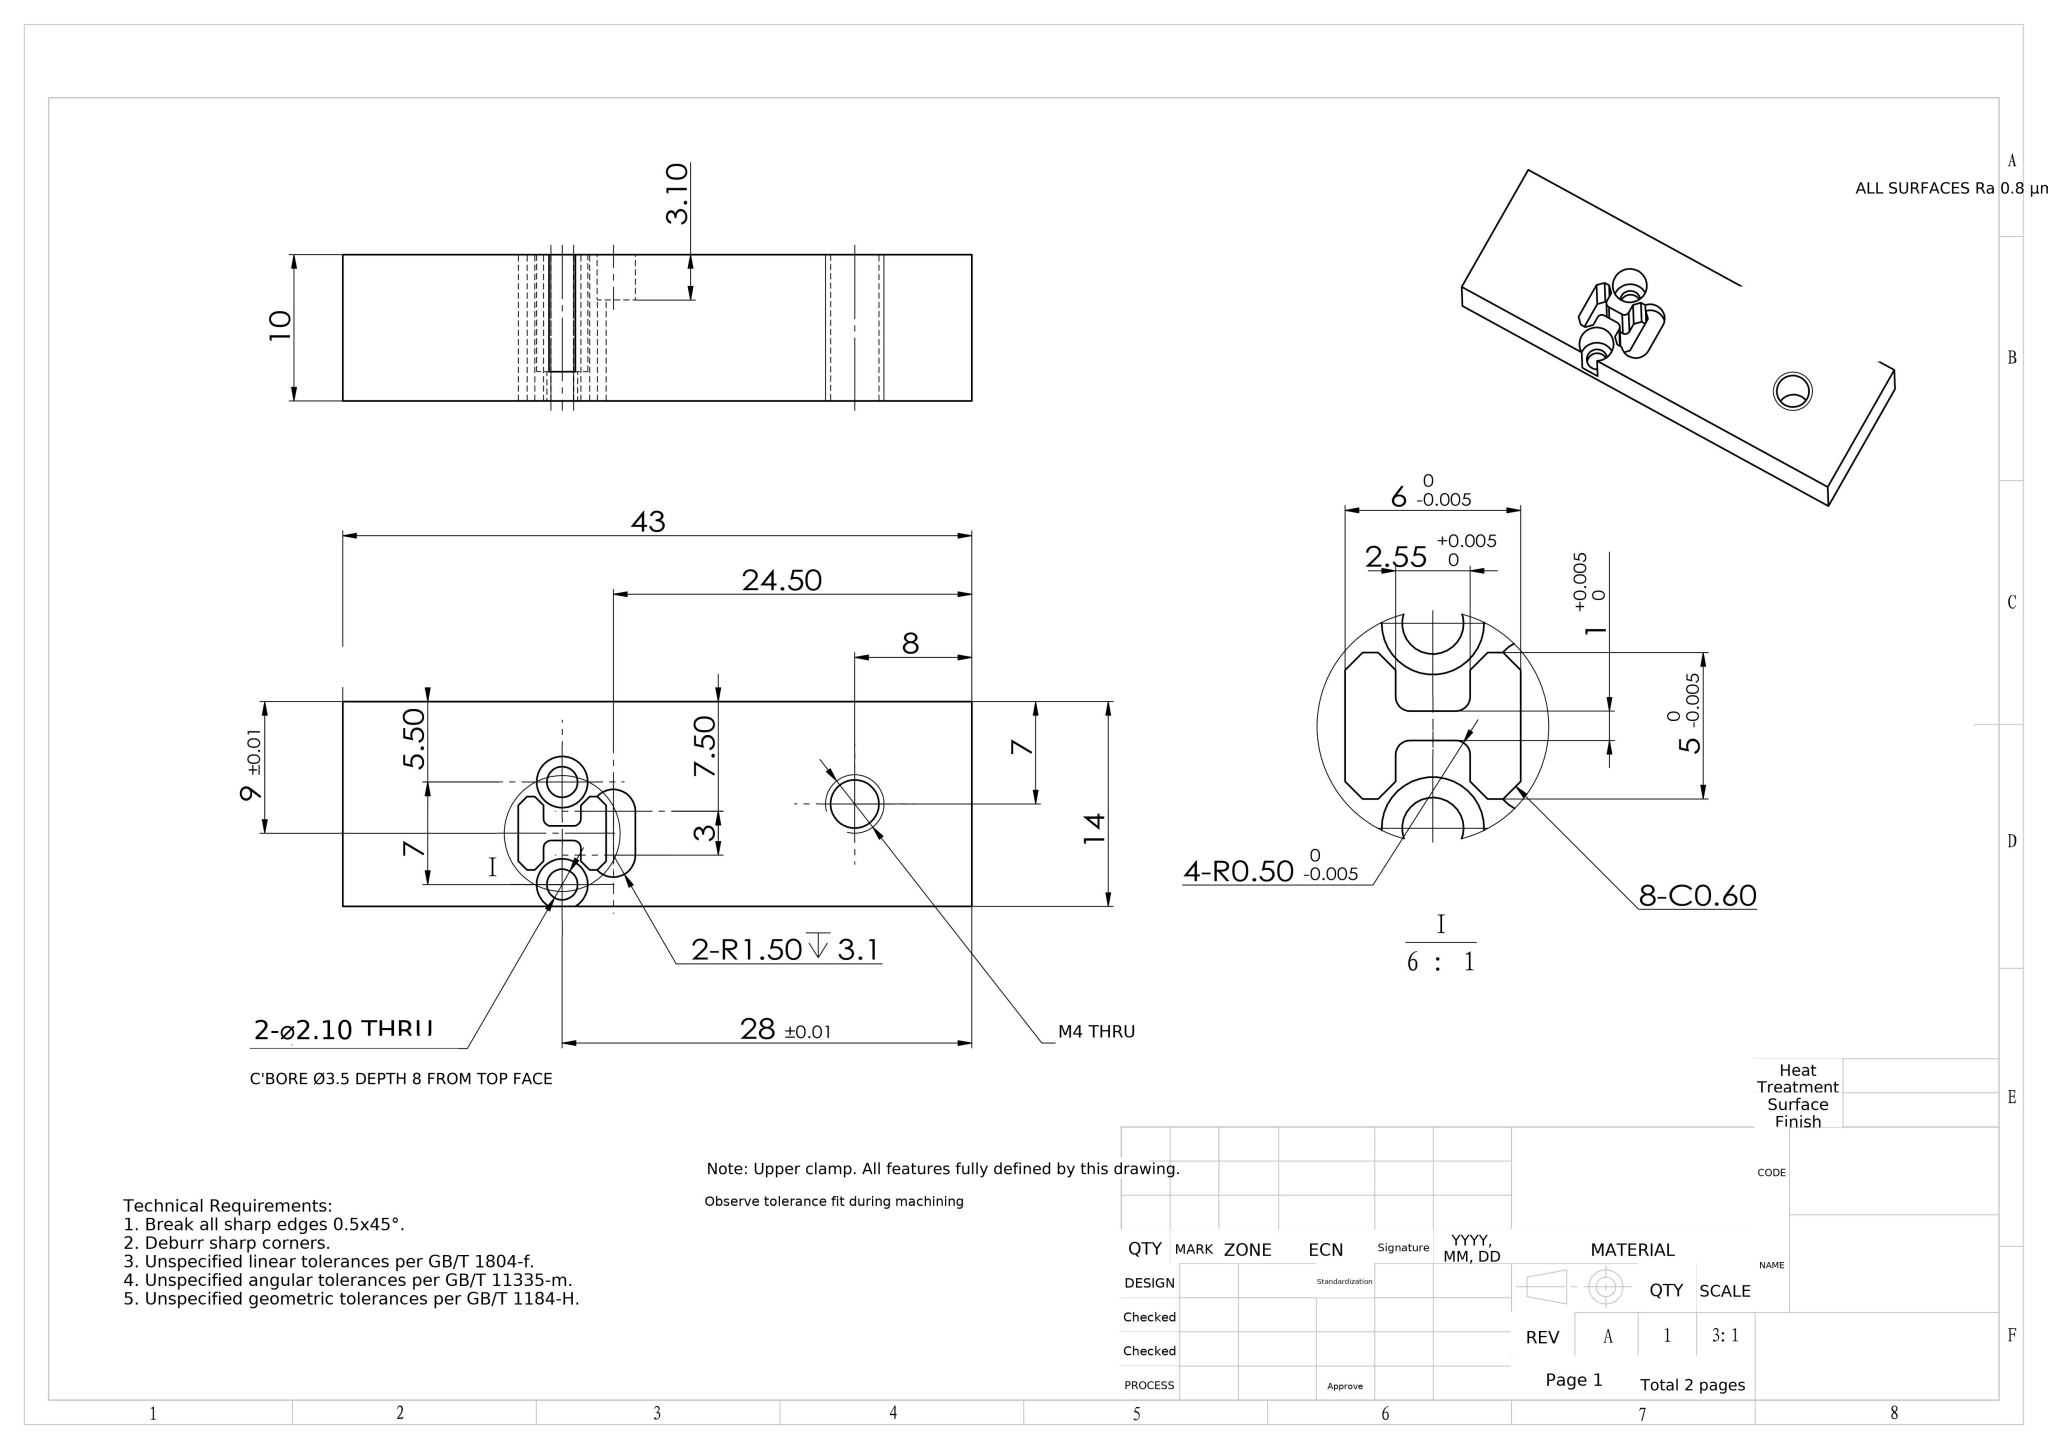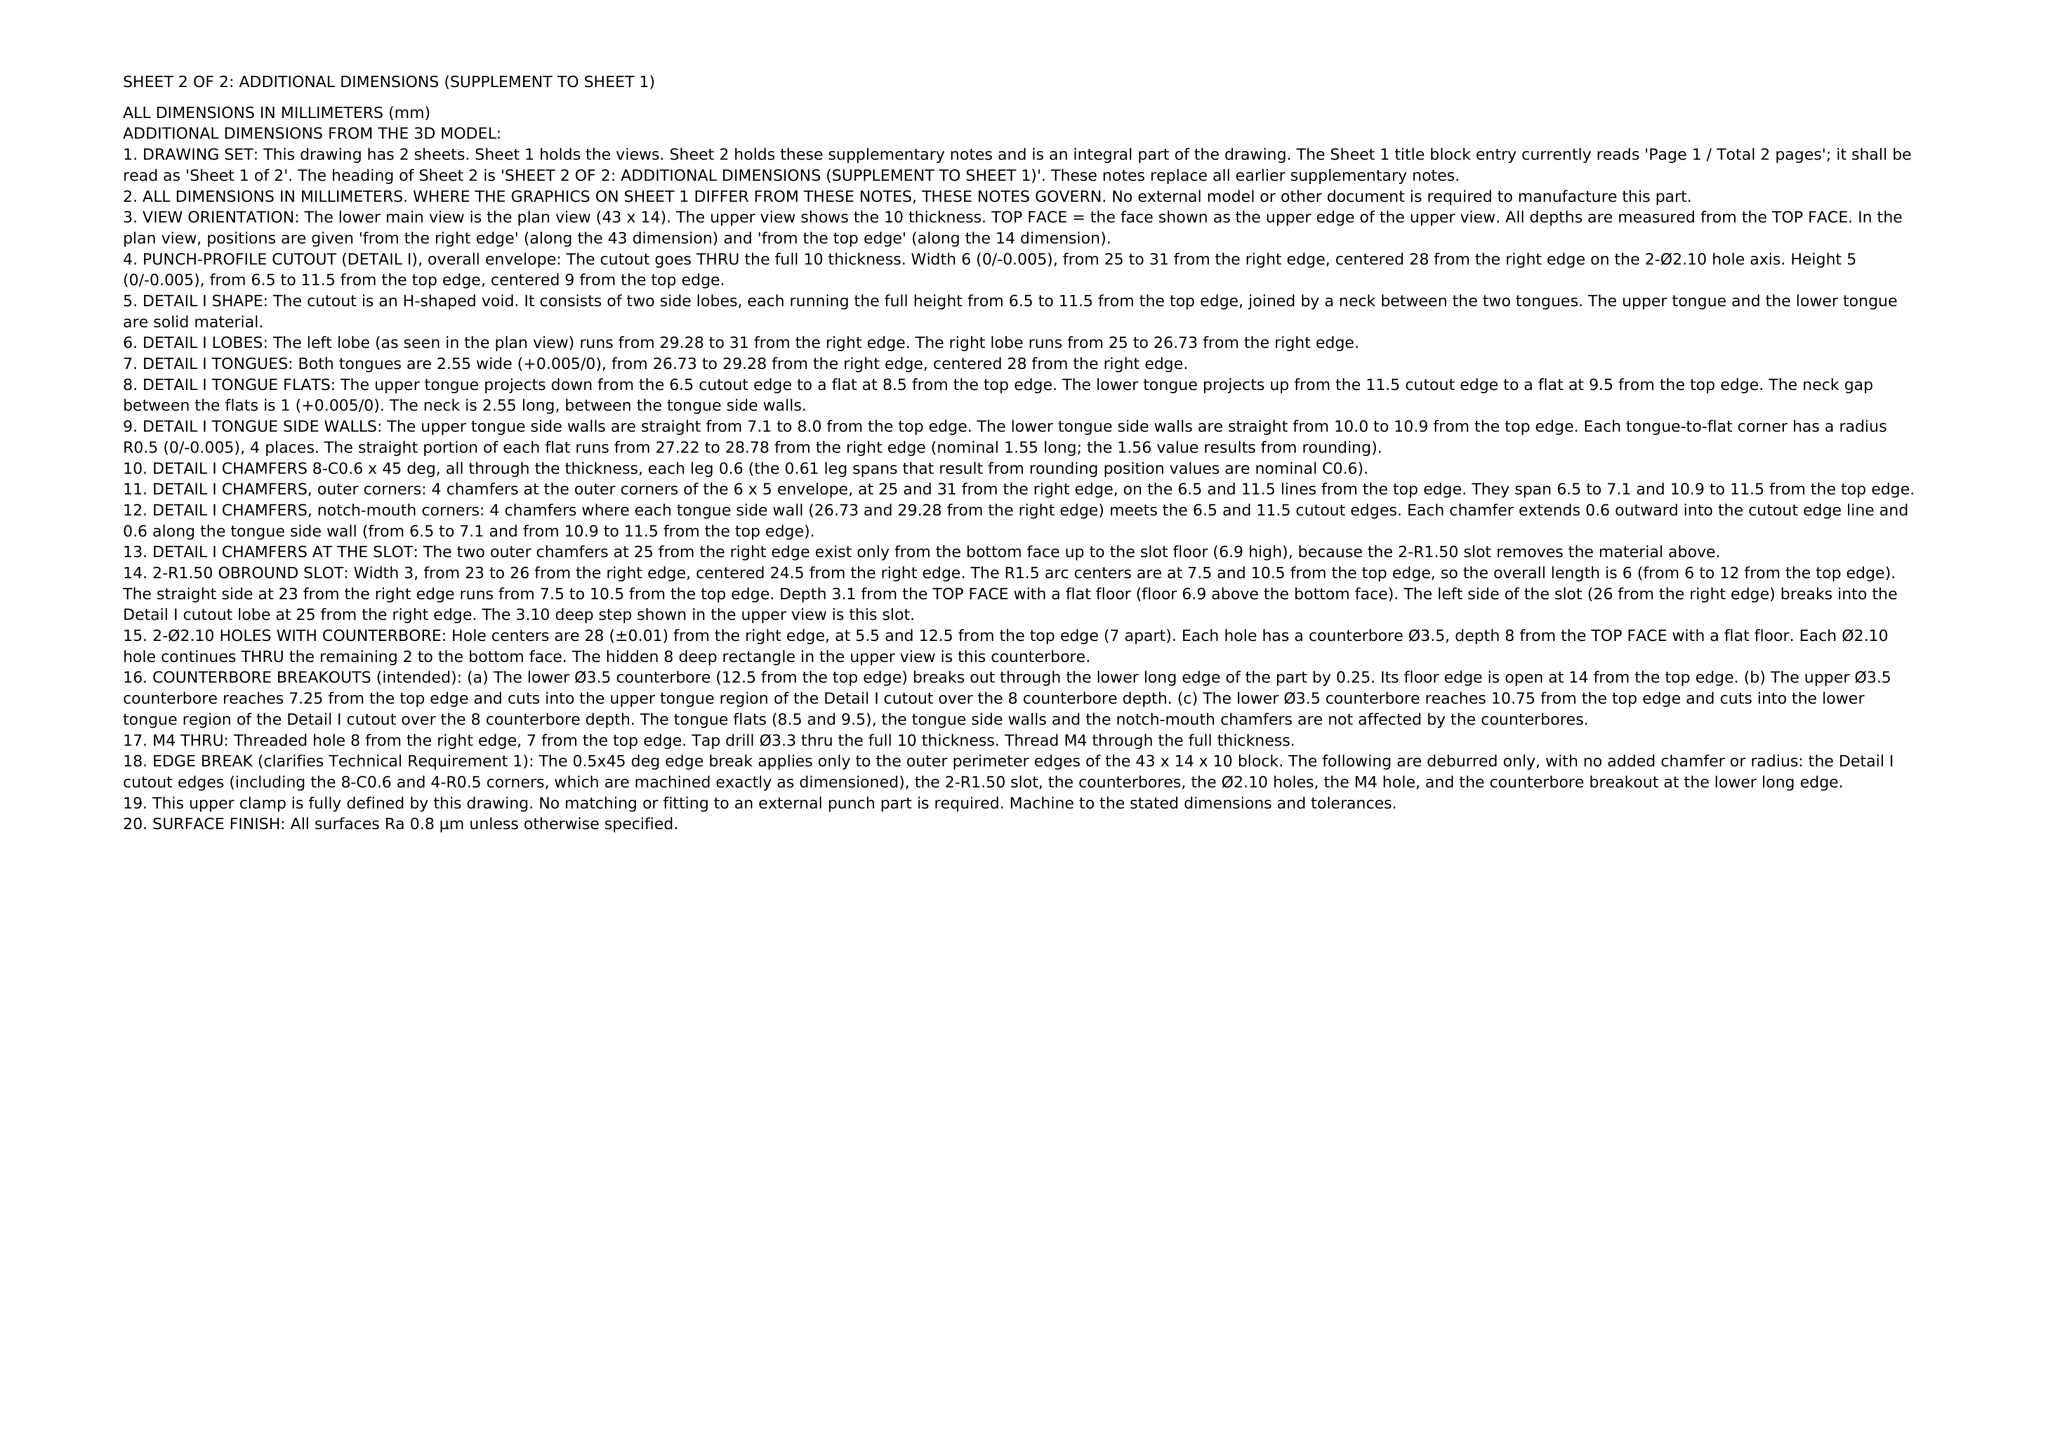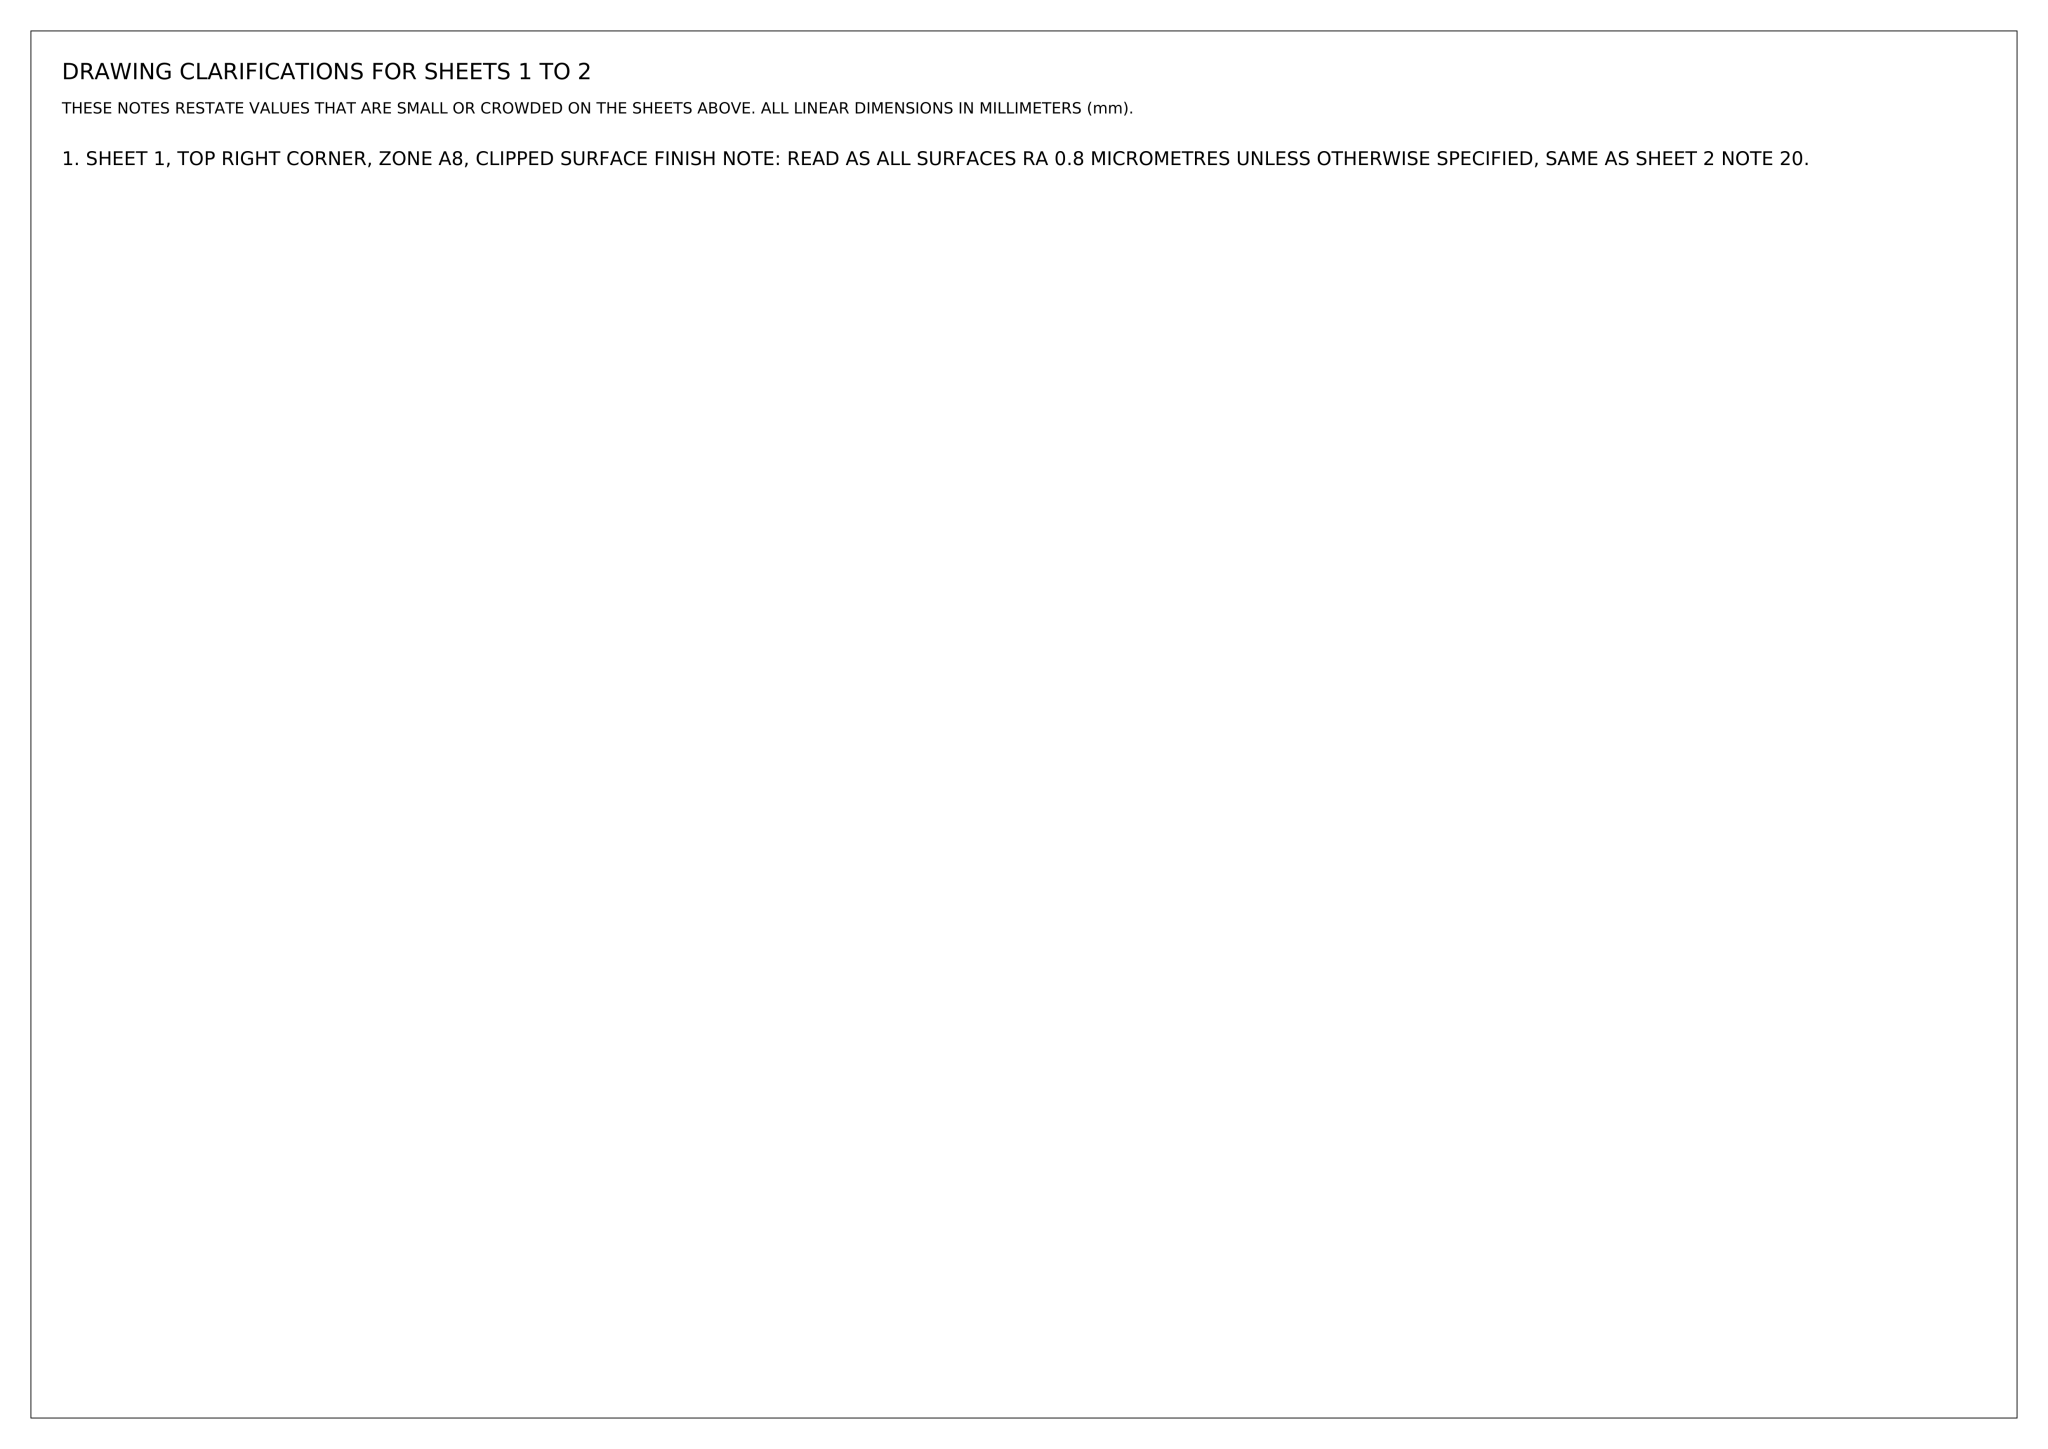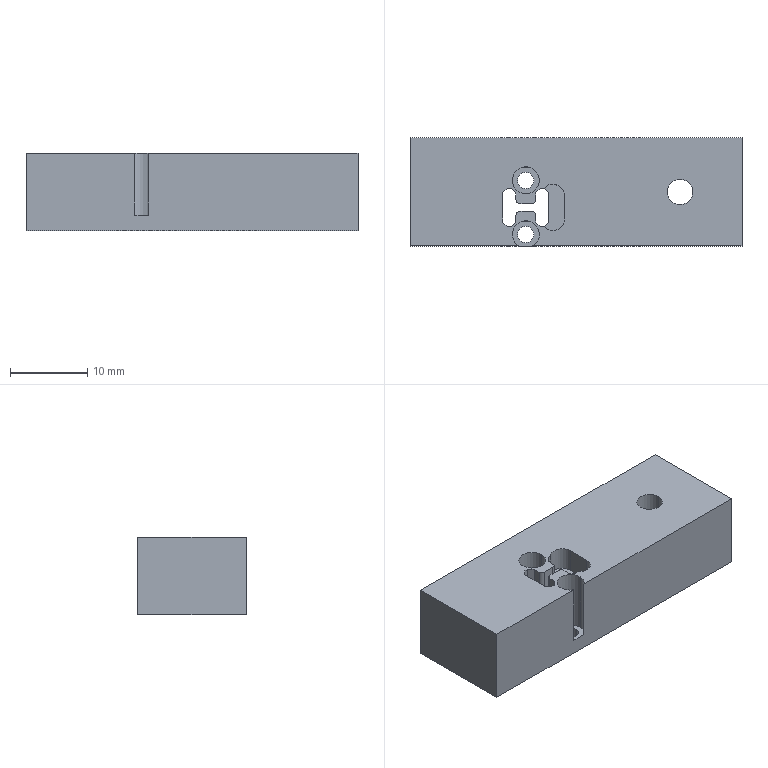Part | NX | mm | Multi-Bore Rectangular Mount Block | 1 solid | 47 faces | box 43 x 14 x 10 mm | volume 5547 mm3 | plane 30 | cylinder 17 | commonest cylinder face diameters 3.5 x5 2.1 x4 1 x4 3.3 x2 3 x2